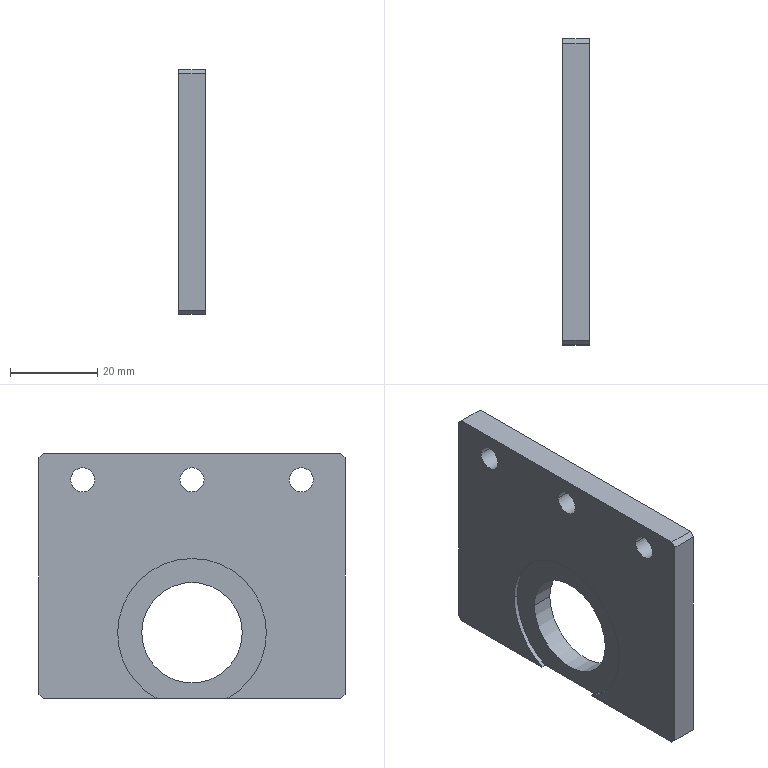Component | SolidWorks | CCDJSTransferCylinderFixingPlate02-1 | 1 solid | 22 faces | box 6 x 70 x 56 mm | volume 20117 mm3 | cylinder 11 | plane 11 | commonest cylinder face diameters 5.5 x6 34 x3 23 x2
build123d program:
from build123d import *

# Parameters (mm, degrees)
SKETCH1_2_W         = 56
SKETCH1_2_H         = 6
BOSS_EXTRUDE1_DEPTH = 30
SKETCH3_W           = 56
SKETCH3_H           = 6
BOSS_EXTRUDE2_DEPTH = 40
SKETCH4_R           = 11.5
CUT_EXTRUDE2_DEPTH  = 25
SKETCH5_R           = 2.75
CUT_EXTRUDE3_DEPTH  = 10
CHAMFER1_SIZE       = 1
SKETCH1_R           = 17
CUT_EXTRUDE1_DEPTH  = 1


with BuildPart() as part:
    # Sketch1_2 → Boss-Extrude1 (new body)
    with BuildSketch(Plane.XY):
        Rectangle(SKETCH1_2_W, SKETCH1_2_H)
    extrude(amount=BOSS_EXTRUDE1_DEPTH)

    # Sketch3 → Boss-Extrude2 (add)
    with BuildSketch(Plane(origin=(0, 0, 0), x_dir=(-1, 0, 0), z_dir=(0, 0, -1))):
        Rectangle(SKETCH3_W, SKETCH3_H)
    extrude(amount=BOSS_EXTRUDE2_DEPTH)

    # Sketch4 → Cut-Extrude2 (cut)
    with BuildSketch(Plane(origin=(0, 3, 0), x_dir=(1, 0, 0), z_dir=(0, 1, 0))):
        with Locations(Location((13, 5, 0), (0, 0, 270))):
            Circle(SKETCH4_R)
    extrude(amount=-CUT_EXTRUDE2_DEPTH, mode=Mode.SUBTRACT)

    # Sketch5 → Cut-Extrude3 (cut)
    with BuildSketch(Plane.XZ.offset(3)):
        with Locations(Location((-22, -5, 0), (0, 0, 270))):
            Circle(SKETCH5_R)
        with Locations(Location((-22, -30, 0), (0, 0, 270))):
            Circle(SKETCH5_R)
        with Locations(Location((-22, 20, 0), (0, 0, 270))):
            Circle(SKETCH5_R)
    extrude(amount=-CUT_EXTRUDE3_DEPTH, mode=Mode.SUBTRACT)

    # Chamfer1
    chamfer1_edges = [part.edges().sort_by_distance(p)[0] for p in [
        (-28, 0, 30),
        (-28, 0, -40),
        (28, 0, -40),
        (28, 0, 30),
    ]]
    chamfer(chamfer1_edges, length=CHAMFER1_SIZE)

    # Sketch1 → Cut-Extrude1 (cut)
    with BuildSketch(Plane(origin=(0, 3, 0), x_dir=(1, 0, 0), z_dir=(0, 1, 0))):
        with Locations((13, 5)):
            Circle(SKETCH1_R)
    extrude(amount=-CUT_EXTRUDE1_DEPTH, mode=Mode.SUBTRACT)


solid = part.part

# Placed as in the assembly
solid = solid.moved(Location((105, 431.564, -50.5), (-90, 0, 90)))
STEP:
#1=COLOUR_RGB('',0.7922,0.8196,0.9333);
#2=FILL_AREA_STYLE_COLOUR('',#1);
#3=FILL_AREA_STYLE('',(#2));
#4=SURFACE_STYLE_FILL_AREA(#3);
#5=SURFACE_SIDE_STYLE('',(#4));
#6=SURFACE_STYLE_USAGE(.BOTH.,#5);
#7=PRESENTATION_STYLE_ASSIGNMENT((#6));
#8=CARTESIAN_POINT('',(4.055,16.125,-2.5));
#9=VERTEX_POINT('',#8);
#10=CARTESIAN_POINT('',(4.055,17.463,-2.5));
#11=VERTEX_POINT('',#10);
#12=CARTESIAN_POINT('',(4.055,16.794,-2.5));
#13=DIRECTION('',(-1.,0.,0.));
#14=DIRECTION('',(0.,1.,0.));
#15=AXIS2_PLACEMENT_3D('',#12,#13,#14);
#16=CIRCLE('',#15,0.6693);
#17=EDGE_CURVE('',#9,#11,#16,.T.);
#18=ORIENTED_EDGE('',*,*,#17,.F.);
#19=CARTESIAN_POINT('',(4.016,16.125,-2.5));
#20=VERTEX_POINT('',#19);
#21=CARTESIAN_POINT('',(4.055,16.125,-2.5));
#22=DIRECTION('',(-1.,0.,0.));
#23=VECTOR('',#22,39.37);
#24=LINE('',#21,#23);
#25=EDGE_CURVE('',#9,#20,#24,.T.);
#26=ORIENTED_EDGE('',*,*,#25,.T.);
#27=CARTESIAN_POINT('',(4.016,17.463,-2.5));
#28=VERTEX_POINT('',#27);
#29=CARTESIAN_POINT('',(4.016,16.794,-2.5));
#30=DIRECTION('',(-1.,0.,0.));
#31=DIRECTION('',(0.,1.,0.));
#32=AXIS2_PLACEMENT_3D('',#29,#30,#31);
#33=CIRCLE('',#32,0.6693);
#34=EDGE_CURVE('',#20,#28,#33,.T.);
#35=ORIENTED_EDGE('',*,*,#34,.T.);
#36=CARTESIAN_POINT('',(4.055,17.463,-2.5));
#37=DIRECTION('',(-1.,0.,0.));
#38=VECTOR('',#37,39.37);
#39=LINE('',#36,#38);
#40=EDGE_CURVE('',#11,#28,#39,.T.);
#41=ORIENTED_EDGE('',*,*,#40,.F.);
#42=EDGE_LOOP('',(#18,#26,#35,#41));
#43=FACE_OUTER_BOUND('',#42,.T.);
#44=CARTESIAN_POINT('',(4.055,16.794,-2.5));
#45=DIRECTION('',(-1.,0.,0.));
#46=DIRECTION('',(0.,1.,0.));
#47=AXIS2_PLACEMENT_3D('',#44,#45,#46);
#48=CYLINDRICAL_SURFACE('',#47,0.6693);
#49=ADVANCED_FACE('',(#43),#48,.F.);
#50=CARTESIAN_POINT('',(4.055,17.109,-3.091));
#51=VERTEX_POINT('',#50);
#52=CARTESIAN_POINT('',(4.055,16.794,-2.5));
#53=DIRECTION('',(-1.,0.,0.));
#54=DIRECTION('',(0.,1.,0.));
#55=AXIS2_PLACEMENT_3D('',#52,#53,#54);
#56=CIRCLE('',#55,0.6693);
#57=EDGE_CURVE('',#11,#51,#56,.T.);
#58=ORIENTED_EDGE('',*,*,#57,.F.);
#59=ORIENTED_EDGE('',*,*,#40,.T.);
#60=CARTESIAN_POINT('',(4.016,17.109,-3.091));
#61=VERTEX_POINT('',#60);
#62=CARTESIAN_POINT('',(4.016,16.794,-2.5));
#63=DIRECTION('',(-1.,0.,0.));
#64=DIRECTION('',(0.,1.,0.));
#65=AXIS2_PLACEMENT_3D('',#62,#63,#64);
#66=CIRCLE('',#65,0.6693);
#67=EDGE_CURVE('',#28,#61,#66,.T.);
#68=ORIENTED_EDGE('',*,*,#67,.T.);
#69=CARTESIAN_POINT('',(4.055,17.109,-3.091));
#70=DIRECTION('',(-1.,0.,0.));
#71=VECTOR('',#70,39.37);
#72=LINE('',#69,#71);
#73=EDGE_CURVE('',#51,#61,#72,.T.);
#74=ORIENTED_EDGE('',*,*,#73,.F.);
#75=EDGE_LOOP('',(#58,#59,#68,#74));
#76=FACE_OUTER_BOUND('',#75,.T.);
#77=CARTESIAN_POINT('',(4.055,16.794,-2.5));
#78=DIRECTION('',(-1.,0.,0.));
#79=DIRECTION('',(0.,1.,0.));
#80=AXIS2_PLACEMENT_3D('',#77,#78,#79);
#81=CYLINDRICAL_SURFACE('',#80,0.6693);
#82=ADVANCED_FACE('',(#76),#81,.F.);
#83=CARTESIAN_POINT('',(4.016,15.918,-1.122));
#84=VERTEX_POINT('',#83);
#85=CARTESIAN_POINT('',(4.016,15.701,-1.122));
#86=VERTEX_POINT('',#85);
#87=CARTESIAN_POINT('',(4.016,15.81,-1.122));
#88=DIRECTION('',(1.,-0.,-0.));
#89=DIRECTION('',(0.,-1.,0.));
#90=AXIS2_PLACEMENT_3D('',#87,#88,#89);
#91=CIRCLE('',#90,0.1083);
#92=EDGE_CURVE('',#84,#86,#91,.T.);
#93=ORIENTED_EDGE('',*,*,#92,.F.);
#94=CARTESIAN_POINT('',(4.252,15.918,-1.122));
#95=VERTEX_POINT('',#94);
#96=CARTESIAN_POINT('',(3.858,15.918,-1.122));
#97=DIRECTION('',(1.,-0.,-0.));
#98=VECTOR('',#97,39.37);
#99=LINE('',#96,#98);
#100=EDGE_CURVE('',#84,#95,#99,.T.);
#101=ORIENTED_EDGE('',*,*,#100,.T.);
#102=CARTESIAN_POINT('',(4.252,15.701,-1.122));
#103=VERTEX_POINT('',#102);
#104=CARTESIAN_POINT('',(4.252,15.81,-1.122));
#105=DIRECTION('',(1.,-0.,-0.));
#106=DIRECTION('',(0.,-1.,0.));
#107=AXIS2_PLACEMENT_3D('',#104,#105,#106);
#108=CIRCLE('',#107,0.1083);
#109=EDGE_CURVE('',#95,#103,#108,.T.);
#110=ORIENTED_EDGE('',*,*,#109,.T.);
#111=CARTESIAN_POINT('',(3.858,15.701,-1.122));
#112=DIRECTION('',(1.,-0.,-0.));
#113=VECTOR('',#112,39.37);
#114=LINE('',#111,#113);
#115=EDGE_CURVE('',#86,#103,#114,.T.);
#116=ORIENTED_EDGE('',*,*,#115,.F.);
#117=EDGE_LOOP('',(#93,#101,#110,#116));
#118=FACE_OUTER_BOUND('',#117,.T.);
#119=CARTESIAN_POINT('',(3.858,15.81,-1.122));
#120=DIRECTION('',(1.,-0.,-0.));
#121=DIRECTION('',(0.,-1.,0.));
#122=AXIS2_PLACEMENT_3D('',#119,#120,#121);
#123=CYLINDRICAL_SURFACE('',#122,0.1083);
#124=ADVANCED_FACE('',(#118),#123,.F.);
#125=CARTESIAN_POINT('',(4.016,17.886,-1.122));
#126=VERTEX_POINT('',#125);
#127=CARTESIAN_POINT('',(4.016,17.67,-1.122));
#128=VERTEX_POINT('',#127);
#129=CARTESIAN_POINT('',(4.016,17.778,-1.122));
#130=DIRECTION('',(1.,-0.,-0.));
#131=DIRECTION('',(0.,-1.,0.));
#132=AXIS2_PLACEMENT_3D('',#129,#130,#131);
#133=CIRCLE('',#132,0.1083);
#134=EDGE_CURVE('',#126,#128,#133,.T.);
#135=ORIENTED_EDGE('',*,*,#134,.F.);
#136=CARTESIAN_POINT('',(4.252,17.886,-1.122));
#137=VERTEX_POINT('',#136);
#138=CARTESIAN_POINT('',(3.858,17.886,-1.122));
#139=DIRECTION('',(1.,-0.,-0.));
#140=VECTOR('',#139,39.37);
#141=LINE('',#138,#140);
#142=EDGE_CURVE('',#126,#137,#141,.T.);
#143=ORIENTED_EDGE('',*,*,#142,.T.);
#144=CARTESIAN_POINT('',(4.252,17.67,-1.122));
#145=VERTEX_POINT('',#144);
#146=CARTESIAN_POINT('',(4.252,17.778,-1.122));
#147=DIRECTION('',(1.,-0.,-0.));
#148=DIRECTION('',(0.,-1.,0.));
#149=AXIS2_PLACEMENT_3D('',#146,#147,#148);
#150=CIRCLE('',#149,0.1083);
#151=EDGE_CURVE('',#137,#145,#150,.T.);
#152=ORIENTED_EDGE('',*,*,#151,.T.);
#153=CARTESIAN_POINT('',(3.858,17.67,-1.122));
#154=DIRECTION('',(1.,-0.,-0.));
#155=VECTOR('',#154,39.37);
#156=LINE('',#153,#155);
#157=EDGE_CURVE('',#128,#145,#156,.T.);
#158=ORIENTED_EDGE('',*,*,#157,.F.);
#159=EDGE_LOOP('',(#135,#143,#152,#158));
#160=FACE_OUTER_BOUND('',#159,.T.);
#161=CARTESIAN_POINT('',(3.858,17.778,-1.122));
#162=DIRECTION('',(1.,-0.,-0.));
#163=DIRECTION('',(0.,-1.,0.));
#164=AXIS2_PLACEMENT_3D('',#161,#162,#163);
#165=CYLINDRICAL_SURFACE('',#164,0.1083);
#166=ADVANCED_FACE('',(#160),#165,.F.);
#167=CARTESIAN_POINT('',(4.016,16.902,-1.122));
#168=VERTEX_POINT('',#167);
#169=CARTESIAN_POINT('',(4.016,16.686,-1.122));
#170=VERTEX_POINT('',#169);
#171=CARTESIAN_POINT('',(4.016,16.794,-1.122));
#172=DIRECTION('',(1.,-0.,-0.));
#173=DIRECTION('',(0.,-1.,0.));
#174=AXIS2_PLACEMENT_3D('',#171,#172,#173);
#175=CIRCLE('',#174,0.1083);
#176=EDGE_CURVE('',#168,#170,#175,.T.);
#177=ORIENTED_EDGE('',*,*,#176,.F.);
#178=CARTESIAN_POINT('',(4.252,16.902,-1.122));
#179=VERTEX_POINT('',#178);
#180=CARTESIAN_POINT('',(3.858,16.902,-1.122));
#181=DIRECTION('',(1.,-0.,-0.));
#182=VECTOR('',#181,39.37);
#183=LINE('',#180,#182);
#184=EDGE_CURVE('',#168,#179,#183,.T.);
#185=ORIENTED_EDGE('',*,*,#184,.T.);
#186=CARTESIAN_POINT('',(4.252,16.686,-1.122));
#187=VERTEX_POINT('',#186);
#188=CARTESIAN_POINT('',(4.252,16.794,-1.122));
#189=DIRECTION('',(1.,-0.,-0.));
#190=DIRECTION('',(0.,-1.,0.));
#191=AXIS2_PLACEMENT_3D('',#188,#189,#190);
#192=CIRCLE('',#191,0.1083);
#193=EDGE_CURVE('',#179,#187,#192,.T.);
#194=ORIENTED_EDGE('',*,*,#193,.T.);
#195=CARTESIAN_POINT('',(3.858,16.686,-1.122));
#196=DIRECTION('',(1.,-0.,-0.));
#197=VECTOR('',#196,39.37);
#198=LINE('',#195,#197);
#199=EDGE_CURVE('',#170,#187,#198,.T.);
#200=ORIENTED_EDGE('',*,*,#199,.F.);
#201=EDGE_LOOP('',(#177,#185,#194,#200));
#202=FACE_OUTER_BOUND('',#201,.T.);
#203=CARTESIAN_POINT('',(3.858,16.794,-1.122));
#204=DIRECTION('',(1.,-0.,-0.));
#205=DIRECTION('',(0.,-1.,0.));
#206=AXIS2_PLACEMENT_3D('',#203,#204,#205);
#207=CYLINDRICAL_SURFACE('',#206,0.1083);
#208=ADVANCED_FACE('',(#202),#207,.F.);
#209=CARTESIAN_POINT('',(4.252,16.341,-2.5));
#210=VERTEX_POINT('',#209);
#211=CARTESIAN_POINT('',(4.252,17.247,-2.5));
#212=VERTEX_POINT('',#211);
#213=CARTESIAN_POINT('',(4.252,16.794,-2.5));
#214=DIRECTION('',(-1.,0.,0.));
#215=DIRECTION('',(0.,1.,0.));
#216=AXIS2_PLACEMENT_3D('',#213,#214,#215);
#217=CIRCLE('',#216,0.4528);
#218=EDGE_CURVE('',#210,#212,#217,.T.);
#219=ORIENTED_EDGE('',*,*,#218,.F.);
#220=CARTESIAN_POINT('',(4.055,16.341,-2.5));
#221=VERTEX_POINT('',#220);
#222=CARTESIAN_POINT('',(5.,16.341,-2.5));
#223=DIRECTION('',(-1.,0.,0.));
#224=VECTOR('',#223,39.37);
#225=LINE('',#222,#224);
#226=EDGE_CURVE('',#210,#221,#225,.T.);
#227=ORIENTED_EDGE('',*,*,#226,.T.);
#228=CARTESIAN_POINT('',(4.055,17.247,-2.5));
#229=VERTEX_POINT('',#228);
#230=CARTESIAN_POINT('',(4.055,16.794,-2.5));
#231=DIRECTION('',(1.,-0.,-0.));
#232=DIRECTION('',(0.,1.,0.));
#233=AXIS2_PLACEMENT_3D('',#230,#231,#232);
#234=CIRCLE('',#233,0.4528);
#235=EDGE_CURVE('',#229,#221,#234,.T.);
#236=ORIENTED_EDGE('',*,*,#235,.F.);
#237=CARTESIAN_POINT('',(5.,17.247,-2.5));
#238=DIRECTION('',(-1.,0.,0.));
#239=VECTOR('',#238,39.37);
#240=LINE('',#237,#239);
#241=EDGE_CURVE('',#212,#229,#240,.T.);
#242=ORIENTED_EDGE('',*,*,#241,.F.);
#243=EDGE_LOOP('',(#219,#227,#236,#242));
#244=FACE_OUTER_BOUND('',#243,.T.);
#245=CARTESIAN_POINT('',(5.,16.794,-2.5));
#246=DIRECTION('',(-1.,0.,0.));
#247=DIRECTION('',(0.,1.,0.));
#248=AXIS2_PLACEMENT_3D('',#245,#246,#247);
#249=CYLINDRICAL_SURFACE('',#248,0.4528);
#250=ADVANCED_FACE('',(#244),#249,.F.);
#251=CARTESIAN_POINT('',(4.016,16.794,-1.122));
#252=DIRECTION('',(1.,-0.,-0.));
#253=DIRECTION('',(0.,-1.,0.));
#254=AXIS2_PLACEMENT_3D('',#251,#252,#253);
#255=CIRCLE('',#254,0.1083);
#256=EDGE_CURVE('',#170,#168,#255,.T.);
#257=ORIENTED_EDGE('',*,*,#256,.T.);
#258=ORIENTED_EDGE('',*,*,#176,.T.);
#259=EDGE_LOOP('',(#257,#258));
#260=FACE_BOUND('',#259,.T.);
#261=CARTESIAN_POINT('',(4.016,17.778,-1.122));
#262=DIRECTION('',(1.,-0.,-0.));
#263=DIRECTION('',(0.,-1.,0.));
#264=AXIS2_PLACEMENT_3D('',#261,#262,#263);
#265=CIRCLE('',#264,0.1083);
#266=EDGE_CURVE('',#128,#126,#265,.T.);
#267=ORIENTED_EDGE('',*,*,#266,.T.);
#268=ORIENTED_EDGE('',*,*,#134,.T.);
#269=EDGE_LOOP('',(#267,#268));
#270=FACE_BOUND('',#269,.T.);
#271=CARTESIAN_POINT('',(4.016,15.81,-1.122));
#272=DIRECTION('',(1.,-0.,-0.));
#273=DIRECTION('',(0.,-1.,0.));
#274=AXIS2_PLACEMENT_3D('',#271,#272,#273);
#275=CIRCLE('',#274,0.1083);
#276=EDGE_CURVE('',#86,#84,#275,.T.);
#277=ORIENTED_EDGE('',*,*,#276,.T.);
#278=ORIENTED_EDGE('',*,*,#92,.T.);
#279=EDGE_LOOP('',(#277,#278));
#280=FACE_BOUND('',#279,.T.);
#281=CARTESIAN_POINT('',(4.016,16.479,-3.091));
#282=VERTEX_POINT('',#281);
#283=CARTESIAN_POINT('',(4.016,16.794,-2.5));
#284=DIRECTION('',(-1.,0.,0.));
#285=DIRECTION('',(0.,1.,0.));
#286=AXIS2_PLACEMENT_3D('',#283,#284,#285);
#287=CIRCLE('',#286,0.6693);
#288=EDGE_CURVE('',#282,#20,#287,.T.);
#289=ORIENTED_EDGE('',*,*,#288,.F.);
#290=CARTESIAN_POINT('',(4.016,15.455,-3.091));
#291=VERTEX_POINT('',#290);
#292=CARTESIAN_POINT('',(4.016,18.172,-3.091));
#293=DIRECTION('',(-0.,-1.,-0.));
#294=VECTOR('',#293,39.37);
#295=LINE('',#292,#294);
#296=EDGE_CURVE('',#282,#291,#295,.T.);
#297=ORIENTED_EDGE('',*,*,#296,.T.);
#298=CARTESIAN_POINT('',(4.016,15.416,-3.051));
#299=VERTEX_POINT('',#298);
#300=CARTESIAN_POINT('',(4.016,15.416,-3.051));
#301=DIRECTION('',(-0.,-0.7071,0.7071));
#302=VECTOR('',#301,39.37);
#303=LINE('',#300,#302);
#304=EDGE_CURVE('',#291,#299,#303,.T.);
#305=ORIENTED_EDGE('',*,*,#304,.T.);
#306=CARTESIAN_POINT('',(4.016,15.416,-0.9252));
#307=VERTEX_POINT('',#306);
#308=CARTESIAN_POINT('',(4.016,15.416,-0.8858));
#309=DIRECTION('',(0.,0.,-1.));
#310=VECTOR('',#309,39.37);
#311=LINE('',#308,#310);
#312=EDGE_CURVE('',#307,#299,#311,.T.);
#313=ORIENTED_EDGE('',*,*,#312,.F.);
#314=CARTESIAN_POINT('',(4.016,15.455,-0.8858));
#315=VERTEX_POINT('',#314);
#316=CARTESIAN_POINT('',(4.016,15.416,-0.9252));
#317=DIRECTION('',(0.,0.7071,0.7071));
#318=VECTOR('',#317,39.37);
#319=LINE('',#316,#318);
#320=EDGE_CURVE('',#307,#315,#319,.T.);
#321=ORIENTED_EDGE('',*,*,#320,.T.);
#322=CARTESIAN_POINT('',(4.016,18.132,-0.8858));
#323=VERTEX_POINT('',#322);
#324=CARTESIAN_POINT('',(4.016,18.172,-0.8858));
#325=DIRECTION('',(-0.,-1.,-0.));
#326=VECTOR('',#325,39.37);
#327=LINE('',#324,#326);
#328=EDGE_CURVE('',#323,#315,#327,.T.);
#329=ORIENTED_EDGE('',*,*,#328,.F.);
#330=CARTESIAN_POINT('',(4.016,18.172,-0.9252));
#331=VERTEX_POINT('',#330);
#332=CARTESIAN_POINT('',(4.016,18.172,-0.9252));
#333=DIRECTION('',(0.,0.7071,-0.7071));
#334=VECTOR('',#333,39.37);
#335=LINE('',#332,#334);
#336=EDGE_CURVE('',#323,#331,#335,.T.);
#337=ORIENTED_EDGE('',*,*,#336,.T.);
#338=CARTESIAN_POINT('',(4.016,18.172,-3.051));
#339=VERTEX_POINT('',#338);
#340=CARTESIAN_POINT('',(4.016,18.172,-0.8858));
#341=DIRECTION('',(0.,-0.,1.));
#342=VECTOR('',#341,39.37);
#343=LINE('',#340,#342);
#344=EDGE_CURVE('',#339,#331,#343,.T.);
#345=ORIENTED_EDGE('',*,*,#344,.F.);
#346=CARTESIAN_POINT('',(4.016,18.132,-3.091));
#347=VERTEX_POINT('',#346);
#348=CARTESIAN_POINT('',(4.016,18.172,-3.051));
#349=DIRECTION('',(-0.,-0.7071,-0.7071));
#350=VECTOR('',#349,39.37);
#351=LINE('',#348,#350);
#352=EDGE_CURVE('',#339,#347,#351,.T.);
#353=ORIENTED_EDGE('',*,*,#352,.T.);
#354=CARTESIAN_POINT('',(4.016,18.172,-3.091));
#355=DIRECTION('',(-0.,-1.,-0.));
#356=VECTOR('',#355,39.37);
#357=LINE('',#354,#356);
#358=EDGE_CURVE('',#347,#61,#357,.T.);
#359=ORIENTED_EDGE('',*,*,#358,.T.);
#360=ORIENTED_EDGE('',*,*,#67,.F.);
#361=ORIENTED_EDGE('',*,*,#34,.F.);
#362=EDGE_LOOP('',(#289,#297,#305,#313,#321,#329,#337,#345,#353,#359,#360,#361));
#363=FACE_OUTER_BOUND('',#362,.T.);
#364=CARTESIAN_POINT('',(4.016,18.172,-0.8858));
#365=DIRECTION('',(1.,-0.,-0.));
#366=DIRECTION('',(-0.,-1.,-0.));
#367=AXIS2_PLACEMENT_3D('',#364,#365,#366);
#368=PLANE('',#367);
#369=ADVANCED_FACE('',(#260,#270,#280,#363),#368,.F.);
#370=ORIENTED_EDGE('',*,*,#226,.F.);
#371=CARTESIAN_POINT('',(4.252,16.794,-2.5));
#372=DIRECTION('',(-1.,0.,0.));
#373=DIRECTION('',(0.,1.,0.));
#374=AXIS2_PLACEMENT_3D('',#371,#372,#373);
#375=CIRCLE('',#374,0.4528);
#376=EDGE_CURVE('',#212,#210,#375,.T.);
#377=ORIENTED_EDGE('',*,*,#376,.F.);
#378=ORIENTED_EDGE('',*,*,#241,.T.);
#379=CARTESIAN_POINT('',(4.055,16.794,-2.5));
#380=DIRECTION('',(1.,-0.,-0.));
#381=DIRECTION('',(0.,1.,0.));
#382=AXIS2_PLACEMENT_3D('',#379,#380,#381);
#383=CIRCLE('',#382,0.4528);
#384=EDGE_CURVE('',#221,#229,#383,.T.);
#385=ORIENTED_EDGE('',*,*,#384,.F.);
#386=EDGE_LOOP('',(#370,#377,#378,#385));
#387=FACE_OUTER_BOUND('',#386,.T.);
#388=CARTESIAN_POINT('',(5.,16.794,-2.5));
#389=DIRECTION('',(-1.,0.,0.));
#390=DIRECTION('',(0.,1.,0.));
#391=AXIS2_PLACEMENT_3D('',#388,#389,#390);
#392=CYLINDRICAL_SURFACE('',#391,0.4528);
#393=ADVANCED_FACE('',(#387),#392,.F.);
#394=CARTESIAN_POINT('',(4.055,16.479,-3.091));
#395=VERTEX_POINT('',#394);
#396=CARTESIAN_POINT('',(4.055,18.172,-3.091));
#397=DIRECTION('',(-0.,-1.,-0.));
#398=VECTOR('',#397,39.37);
#399=LINE('',#396,#398);
#400=EDGE_CURVE('',#51,#395,#399,.T.);
#401=ORIENTED_EDGE('',*,*,#400,.F.);
#402=ORIENTED_EDGE('',*,*,#73,.T.);
#403=ORIENTED_EDGE('',*,*,#358,.F.);
#404=CARTESIAN_POINT('',(4.252,18.132,-3.091));
#405=VERTEX_POINT('',#404);
#406=CARTESIAN_POINT('',(4.252,18.132,-3.091));
#407=DIRECTION('',(1.,-0.,-0.));
#408=VECTOR('',#407,39.37);
#409=LINE('',#406,#408);
#410=EDGE_CURVE('',#347,#405,#409,.T.);
#411=ORIENTED_EDGE('',*,*,#410,.T.);
#412=CARTESIAN_POINT('',(4.252,15.455,-3.091));
#413=VERTEX_POINT('',#412);
#414=CARTESIAN_POINT('',(4.252,18.172,-3.091));
#415=DIRECTION('',(-0.,-1.,-0.));
#416=VECTOR('',#415,39.37);
#417=LINE('',#414,#416);
#418=EDGE_CURVE('',#405,#413,#417,.T.);
#419=ORIENTED_EDGE('',*,*,#418,.T.);
#420=CARTESIAN_POINT('',(4.252,15.455,-3.091));
#421=DIRECTION('',(-1.,0.,0.));
#422=VECTOR('',#421,39.37);
#423=LINE('',#420,#422);
#424=EDGE_CURVE('',#413,#291,#423,.T.);
#425=ORIENTED_EDGE('',*,*,#424,.T.);
#426=ORIENTED_EDGE('',*,*,#296,.F.);
#427=CARTESIAN_POINT('',(4.055,16.479,-3.091));
#428=DIRECTION('',(1.,-0.,-0.));
#429=VECTOR('',#428,39.37);
#430=LINE('',#427,#429);
#431=EDGE_CURVE('',#282,#395,#430,.T.);
#432=ORIENTED_EDGE('',*,*,#431,.T.);
#433=EDGE_LOOP('',(#401,#402,#403,#411,#419,#425,#426,#432));
#434=FACE_OUTER_BOUND('',#433,.T.);
#435=CARTESIAN_POINT('',(4.252,18.172,-3.091));
#436=DIRECTION('',(0.,-0.,1.));
#437=DIRECTION('',(0.,1.,0.));
#438=AXIS2_PLACEMENT_3D('',#435,#436,#437);
#439=PLANE('',#438);
#440=ADVANCED_FACE('',(#434),#439,.F.);
#441=CARTESIAN_POINT('',(4.252,18.132,-0.8858));
#442=VERTEX_POINT('',#441);
#443=CARTESIAN_POINT('',(4.252,15.455,-0.8858));
#444=VERTEX_POINT('',#443);
#445=CARTESIAN_POINT('',(4.252,18.172,-0.8858));
#446=DIRECTION('',(-0.,-1.,-0.));
#447=VECTOR('',#446,39.37);
#448=LINE('',#445,#447);
#449=EDGE_CURVE('',#442,#444,#448,.T.);
#450=ORIENTED_EDGE('',*,*,#449,.F.);
#451=CARTESIAN_POINT('',(4.252,18.132,-0.8858));
#452=DIRECTION('',(-1.,0.,0.));
#453=VECTOR('',#452,39.37);
#454=LINE('',#451,#453);
#455=EDGE_CURVE('',#442,#323,#454,.T.);
#456=ORIENTED_EDGE('',*,*,#455,.T.);
#457=ORIENTED_EDGE('',*,*,#328,.T.);
#458=CARTESIAN_POINT('',(4.252,15.455,-0.8858));
#459=DIRECTION('',(1.,-0.,-0.));
#460=VECTOR('',#459,39.37);
#461=LINE('',#458,#460);
#462=EDGE_CURVE('',#315,#444,#461,.T.);
#463=ORIENTED_EDGE('',*,*,#462,.T.);
#464=EDGE_LOOP('',(#450,#456,#457,#463));
#465=FACE_OUTER_BOUND('',#464,.T.);
#466=CARTESIAN_POINT('',(4.252,18.172,-0.8858));
#467=DIRECTION('',(-0.,0.,-1.));
#468=DIRECTION('',(-0.,-1.,-0.));
#469=AXIS2_PLACEMENT_3D('',#466,#467,#468);
#470=PLANE('',#469);
#471=ADVANCED_FACE('',(#465),#470,.F.);
#472=CARTESIAN_POINT('',(4.252,15.81,-1.122));
#473=DIRECTION('',(1.,-0.,-0.));
#474=DIRECTION('',(0.,-1.,0.));
#475=AXIS2_PLACEMENT_3D('',#472,#473,#474);
#476=CIRCLE('',#475,0.1083);
#477=EDGE_CURVE('',#103,#95,#476,.T.);
#478=ORIENTED_EDGE('',*,*,#477,.F.);
#479=ORIENTED_EDGE('',*,*,#109,.F.);
#480=EDGE_LOOP('',(#478,#479));
#481=FACE_BOUND('',#480,.T.);
#482=CARTESIAN_POINT('',(4.252,17.778,-1.122));
#483=DIRECTION('',(1.,-0.,-0.));
#484=DIRECTION('',(0.,-1.,0.));
#485=AXIS2_PLACEMENT_3D('',#482,#483,#484);
#486=CIRCLE('',#485,0.1083);
#487=EDGE_CURVE('',#145,#137,#486,.T.);
#488=ORIENTED_EDGE('',*,*,#487,.F.);
#489=ORIENTED_EDGE('',*,*,#151,.F.);
#490=EDGE_LOOP('',(#488,#489));
#491=FACE_BOUND('',#490,.T.);
#492=CARTESIAN_POINT('',(4.252,16.794,-1.122));
#493=DIRECTION('',(1.,-0.,-0.));
#494=DIRECTION('',(0.,-1.,0.));
#495=AXIS2_PLACEMENT_3D('',#492,#493,#494);
#496=CIRCLE('',#495,0.1083);
#497=EDGE_CURVE('',#187,#179,#496,.T.);
#498=ORIENTED_EDGE('',*,*,#497,.F.);
#499=ORIENTED_EDGE('',*,*,#193,.F.);
#500=EDGE_LOOP('',(#498,#499));
#501=FACE_BOUND('',#500,.T.);
#502=ORIENTED_EDGE('',*,*,#376,.T.);
#503=ORIENTED_EDGE('',*,*,#218,.T.);
#504=EDGE_LOOP('',(#502,#503));
#505=FACE_BOUND('',#504,.T.);
#506=CARTESIAN_POINT('',(4.252,18.172,-0.9252));
#507=VERTEX_POINT('',#506);
#508=CARTESIAN_POINT('',(4.252,18.172,-3.051));
#509=VERTEX_POINT('',#508);
#510=CARTESIAN_POINT('',(4.252,18.172,-0.8858));
#511=DIRECTION('',(-0.,0.,-1.));
#512=VECTOR('',#511,39.37);
#513=LINE('',#510,#512);
#514=EDGE_CURVE('',#507,#509,#513,.T.);
#515=ORIENTED_EDGE('',*,*,#514,.F.);
#516=CARTESIAN_POINT('',(4.252,18.172,-0.9252));
#517=DIRECTION('',(-0.,-0.7071,0.7071));
#518=VECTOR('',#517,39.37);
#519=LINE('',#516,#518);
#520=EDGE_CURVE('',#507,#442,#519,.T.);
#521=ORIENTED_EDGE('',*,*,#520,.T.);
#522=ORIENTED_EDGE('',*,*,#449,.T.);
#523=CARTESIAN_POINT('',(4.252,15.416,-0.9252));
#524=VERTEX_POINT('',#523);
#525=CARTESIAN_POINT('',(4.252,15.416,-0.9252));
#526=DIRECTION('',(-0.,-0.7071,-0.7071));
#527=VECTOR('',#526,39.37);
#528=LINE('',#525,#527);
#529=EDGE_CURVE('',#444,#524,#528,.T.);
#530=ORIENTED_EDGE('',*,*,#529,.T.);
#531=CARTESIAN_POINT('',(4.252,15.416,-3.051));
#532=VERTEX_POINT('',#531);
#533=CARTESIAN_POINT('',(4.252,15.416,-0.8858));
#534=DIRECTION('',(-0.,-0.,1.));
#535=VECTOR('',#534,39.37);
#536=LINE('',#533,#535);
#537=EDGE_CURVE('',#532,#524,#536,.T.);
#538=ORIENTED_EDGE('',*,*,#537,.F.);
#539=CARTESIAN_POINT('',(4.252,15.416,-3.051));
#540=DIRECTION('',(0.,0.7071,-0.7071));
#541=VECTOR('',#540,39.37);
#542=LINE('',#539,#541);
#543=EDGE_CURVE('',#532,#413,#542,.T.);
#544=ORIENTED_EDGE('',*,*,#543,.T.);
#545=ORIENTED_EDGE('',*,*,#418,.F.);
#546=CARTESIAN_POINT('',(4.252,18.172,-3.051));
#547=DIRECTION('',(0.,0.7071,0.7071));
#548=VECTOR('',#547,39.37);
#549=LINE('',#546,#548);
#550=EDGE_CURVE('',#405,#509,#549,.T.);
#551=ORIENTED_EDGE('',*,*,#550,.T.);
#552=EDGE_LOOP('',(#515,#521,#522,#530,#538,#544,#545,#551));
#553=FACE_OUTER_BOUND('',#552,.T.);
#554=CARTESIAN_POINT('',(4.252,18.172,-0.8858));
#555=DIRECTION('',(-1.,0.,0.));
#556=DIRECTION('',(0.,1.,0.));
#557=AXIS2_PLACEMENT_3D('',#554,#555,#556);
#558=PLANE('',#557);
#559=ADVANCED_FACE('',(#481,#491,#501,#505,#553),#558,.F.);
#560=ORIENTED_EDGE('',*,*,#344,.T.);
#561=CARTESIAN_POINT('',(4.134,18.172,-0.9252));
#562=DIRECTION('',(1.,-0.,-0.));
#563=VECTOR('',#562,39.37);
#564=LINE('',#561,#563);
#565=EDGE_CURVE('',#331,#507,#564,.T.);
#566=ORIENTED_EDGE('',*,*,#565,.T.);
#567=ORIENTED_EDGE('',*,*,#514,.T.);
#568=CARTESIAN_POINT('',(4.134,18.172,-3.051));
#569=DIRECTION('',(-1.,0.,0.));
#570=VECTOR('',#569,39.37);
#571=LINE('',#568,#570);
#572=EDGE_CURVE('',#509,#339,#571,.T.);
#573=ORIENTED_EDGE('',*,*,#572,.T.);
#574=EDGE_LOOP('',(#560,#566,#567,#573));
#575=FACE_OUTER_BOUND('',#574,.T.);
#576=CARTESIAN_POINT('',(4.134,18.172,-1.988));
#577=DIRECTION('',(-0.,-1.,-0.));
#578=DIRECTION('',(0.,-0.,1.));
#579=AXIS2_PLACEMENT_3D('',#576,#577,#578);
#580=PLANE('',#579);
#581=ADVANCED_FACE('',(#575),#580,.F.);
#582=ORIENTED_EDGE('',*,*,#312,.T.);
#583=CARTESIAN_POINT('',(4.134,15.416,-3.051));
#584=DIRECTION('',(1.,-0.,-0.));
#585=VECTOR('',#584,39.37);
#586=LINE('',#583,#585);
#587=EDGE_CURVE('',#299,#532,#586,.T.);
#588=ORIENTED_EDGE('',*,*,#587,.T.);
#589=ORIENTED_EDGE('',*,*,#537,.T.);
#590=CARTESIAN_POINT('',(4.134,15.416,-0.9252));
#591=DIRECTION('',(-1.,0.,0.));
#592=VECTOR('',#591,39.37);
#593=LINE('',#590,#592);
#594=EDGE_CURVE('',#524,#307,#593,.T.);
#595=ORIENTED_EDGE('',*,*,#594,.T.);
#596=EDGE_LOOP('',(#582,#588,#589,#595));
#597=FACE_OUTER_BOUND('',#596,.T.);
#598=CARTESIAN_POINT('',(4.134,15.416,-1.988));
#599=DIRECTION('',(0.,1.,0.));
#600=DIRECTION('',(-0.,0.,-1.));
#601=AXIS2_PLACEMENT_3D('',#598,#599,#600);
#602=PLANE('',#601);
#603=ADVANCED_FACE('',(#597),#602,.F.);
#604=ORIENTED_EDGE('',*,*,#184,.F.);
#605=ORIENTED_EDGE('',*,*,#256,.F.);
#606=ORIENTED_EDGE('',*,*,#199,.T.);
#607=ORIENTED_EDGE('',*,*,#497,.T.);
#608=EDGE_LOOP('',(#604,#605,#606,#607));
#609=FACE_OUTER_BOUND('',#608,.T.);
#610=CARTESIAN_POINT('',(3.858,16.794,-1.122));
#611=DIRECTION('',(1.,-0.,-0.));
#612=DIRECTION('',(0.,-1.,0.));
#613=AXIS2_PLACEMENT_3D('',#610,#611,#612);
#614=CYLINDRICAL_SURFACE('',#613,0.1083);
#615=ADVANCED_FACE('',(#609),#614,.F.);
#616=ORIENTED_EDGE('',*,*,#142,.F.);
#617=ORIENTED_EDGE('',*,*,#266,.F.);
#618=ORIENTED_EDGE('',*,*,#157,.T.);
#619=ORIENTED_EDGE('',*,*,#487,.T.);
#620=EDGE_LOOP('',(#616,#617,#618,#619));
#621=FACE_OUTER_BOUND('',#620,.T.);
#622=CARTESIAN_POINT('',(3.858,17.778,-1.122));
#623=DIRECTION('',(1.,-0.,-0.));
#624=DIRECTION('',(0.,-1.,0.));
#625=AXIS2_PLACEMENT_3D('',#622,#623,#624);
#626=CYLINDRICAL_SURFACE('',#625,0.1083);
#627=ADVANCED_FACE('',(#621),#626,.F.);
#628=ORIENTED_EDGE('',*,*,#100,.F.);
#629=ORIENTED_EDGE('',*,*,#276,.F.);
#630=ORIENTED_EDGE('',*,*,#115,.T.);
#631=ORIENTED_EDGE('',*,*,#477,.T.);
#632=EDGE_LOOP('',(#628,#629,#630,#631));
#633=FACE_OUTER_BOUND('',#632,.T.);
#634=CARTESIAN_POINT('',(3.858,15.81,-1.122));
#635=DIRECTION('',(1.,-0.,-0.));
#636=DIRECTION('',(0.,-1.,0.));
#637=AXIS2_PLACEMENT_3D('',#634,#635,#636);
#638=CYLINDRICAL_SURFACE('',#637,0.1083);
#639=ADVANCED_FACE('',(#633),#638,.F.);
#640=ORIENTED_EDGE('',*,*,#336,.F.);
#641=ORIENTED_EDGE('',*,*,#455,.F.);
#642=ORIENTED_EDGE('',*,*,#520,.F.);
#643=ORIENTED_EDGE('',*,*,#565,.F.);
#644=EDGE_LOOP('',(#640,#641,#642,#643));
#645=FACE_OUTER_BOUND('',#644,.T.);
#646=CARTESIAN_POINT('',(4.134,18.172,-0.9252));
#647=DIRECTION('',(-0.,-0.7071,-0.7071));
#648=DIRECTION('',(1.,-0.,-0.));
#649=AXIS2_PLACEMENT_3D('',#646,#647,#648);
#650=PLANE('',#649);
#651=ADVANCED_FACE('',(#645),#650,.F.);
#652=ORIENTED_EDGE('',*,*,#550,.F.);
#653=ORIENTED_EDGE('',*,*,#410,.F.);
#654=ORIENTED_EDGE('',*,*,#352,.F.);
#655=ORIENTED_EDGE('',*,*,#572,.F.);
#656=EDGE_LOOP('',(#652,#653,#654,#655));
#657=FACE_OUTER_BOUND('',#656,.T.);
#658=CARTESIAN_POINT('',(4.134,18.172,-3.051));
#659=DIRECTION('',(-0.,-0.7071,0.7071));
#660=DIRECTION('',(-1.,0.,0.));
#661=AXIS2_PLACEMENT_3D('',#658,#659,#660);
#662=PLANE('',#661);
#663=ADVANCED_FACE('',(#657),#662,.F.);
#664=ORIENTED_EDGE('',*,*,#304,.F.);
#665=ORIENTED_EDGE('',*,*,#424,.F.);
#666=ORIENTED_EDGE('',*,*,#543,.F.);
#667=ORIENTED_EDGE('',*,*,#587,.F.);
#668=EDGE_LOOP('',(#664,#665,#666,#667));
#669=FACE_OUTER_BOUND('',#668,.T.);
#670=CARTESIAN_POINT('',(4.134,15.416,-3.051));
#671=DIRECTION('',(0.,0.7071,0.7071));
#672=DIRECTION('',(1.,-0.,-0.));
#673=AXIS2_PLACEMENT_3D('',#670,#671,#672);
#674=PLANE('',#673);
#675=ADVANCED_FACE('',(#669),#674,.F.);
#676=ORIENTED_EDGE('',*,*,#529,.F.);
#677=ORIENTED_EDGE('',*,*,#462,.F.);
#678=ORIENTED_EDGE('',*,*,#320,.F.);
#679=ORIENTED_EDGE('',*,*,#594,.F.);
#680=EDGE_LOOP('',(#676,#677,#678,#679));
#681=FACE_OUTER_BOUND('',#680,.T.);
#682=CARTESIAN_POINT('',(4.134,15.416,-0.9252));
#683=DIRECTION('',(0.,0.7071,-0.7071));
#684=DIRECTION('',(-1.,0.,0.));
#685=AXIS2_PLACEMENT_3D('',#682,#683,#684);
#686=PLANE('',#685);
#687=ADVANCED_FACE('',(#681),#686,.F.);
#688=ORIENTED_EDGE('',*,*,#25,.F.);
#689=CARTESIAN_POINT('',(4.055,16.794,-2.5));
#690=DIRECTION('',(-1.,0.,0.));
#691=DIRECTION('',(0.,1.,0.));
#692=AXIS2_PLACEMENT_3D('',#689,#690,#691);
#693=CIRCLE('',#692,0.6693);
#694=EDGE_CURVE('',#395,#9,#693,.T.);
#695=ORIENTED_EDGE('',*,*,#694,.F.);
#696=ORIENTED_EDGE('',*,*,#431,.F.);
#697=ORIENTED_EDGE('',*,*,#288,.T.);
#698=EDGE_LOOP('',(#688,#695,#696,#697));
#699=FACE_OUTER_BOUND('',#698,.T.);
#700=CARTESIAN_POINT('',(4.055,16.794,-2.5));
#701=DIRECTION('',(-1.,0.,0.));
#702=DIRECTION('',(0.,1.,0.));
#703=AXIS2_PLACEMENT_3D('',#700,#701,#702);
#704=CYLINDRICAL_SURFACE('',#703,0.6693);
#705=ADVANCED_FACE('',(#699),#704,.F.);
#706=ORIENTED_EDGE('',*,*,#235,.T.);
#707=ORIENTED_EDGE('',*,*,#384,.T.);
#708=EDGE_LOOP('',(#706,#707));
#709=FACE_BOUND('',#708,.T.);
#710=ORIENTED_EDGE('',*,*,#400,.T.);
#711=ORIENTED_EDGE('',*,*,#694,.T.);
#712=ORIENTED_EDGE('',*,*,#17,.T.);
#713=ORIENTED_EDGE('',*,*,#57,.T.);
#714=EDGE_LOOP('',(#710,#711,#712,#713));
#715=FACE_OUTER_BOUND('',#714,.T.);
#716=CARTESIAN_POINT('',(4.055,16.794,-2.5));
#717=DIRECTION('',(-1.,0.,0.));
#718=DIRECTION('',(0.,1.,0.));
#719=AXIS2_PLACEMENT_3D('',#716,#717,#718);
#720=PLANE('',#719);
#721=ADVANCED_FACE('',(#709,#715),#720,.T.);
#722=CLOSED_SHELL('',(#49,#82,#124,#166,#208,#250,#369,#393,#440,#471,#559,#581,#603,#615,#627,#639,#651,#663,#675,#687,#705,#721));
#723=MANIFOLD_SOLID_BREP('',#722);
#724=STYLED_ITEM('',(#7),#723);
#725=PRESENTATION_LAYER_ASSIGNMENT('','',(#724));
#726=CARTESIAN_POINT('',(0.,0.,0.));
#727=DIRECTION('',(0.,0.,1.));
#728=DIRECTION('',(1.,0.,0.));
#729=AXIS2_PLACEMENT_3D('',#726,#727,#728);
#730=(LENGTH_UNIT()NAMED_UNIT(*)SI_UNIT($,.METRE.));
#731=LENGTH_MEASURE_WITH_UNIT(LENGTH_MEASURE(0.0254),#730);
#732=DIMENSIONAL_EXPONENTS(1.,0.,0.,0.,0.,0.,0.);
#733=(CONVERSION_BASED_UNIT('',#731)LENGTH_UNIT()NAMED_UNIT(#732));
#734=UNCERTAINTY_MEASURE_WITH_UNIT(LENGTH_MEASURE(0.00001),#733,'','');
#735=(NAMED_UNIT(*)PLANE_ANGLE_UNIT()SI_UNIT($,.RADIAN.));
#736=(NAMED_UNIT(*)SI_UNIT($,.STERADIAN.)SOLID_ANGLE_UNIT());
#737=(GEOMETRIC_REPRESENTATION_CONTEXT(3)GLOBAL_UNCERTAINTY_ASSIGNED_CONTEXT((#734))GLOBAL_UNIT_ASSIGNED_CONTEXT((#733,#735,#736))REPRESENTATION_CONTEXT('',''));
#738=ADVANCED_BREP_SHAPE_REPRESENTATION('',(#723,#729),#737);
#739=(LENGTH_UNIT()NAMED_UNIT(*)SI_UNIT($,.METRE.));
#740=LENGTH_MEASURE_WITH_UNIT(LENGTH_MEASURE(0.0254),#739);
#741=DIMENSIONAL_EXPONENTS(1.,0.,0.,0.,0.,0.,0.);
#742=(CONVERSION_BASED_UNIT('',#740)LENGTH_UNIT()NAMED_UNIT(#741));
#743=UNCERTAINTY_MEASURE_WITH_UNIT(LENGTH_MEASURE(0.00001),#742,'','');
#744=(NAMED_UNIT(*)PLANE_ANGLE_UNIT()SI_UNIT($,.RADIAN.));
#745=(NAMED_UNIT(*)SI_UNIT($,.STERADIAN.)SOLID_ANGLE_UNIT());
#746=(GEOMETRIC_REPRESENTATION_CONTEXT(3)GLOBAL_UNCERTAINTY_ASSIGNED_CONTEXT((#743))GLOBAL_UNIT_ASSIGNED_CONTEXT((#742,#744,#745))REPRESENTATION_CONTEXT('',''));
#747=MECHANICAL_DESIGN_GEOMETRIC_PRESENTATION_REPRESENTATION('',(#724),#746);